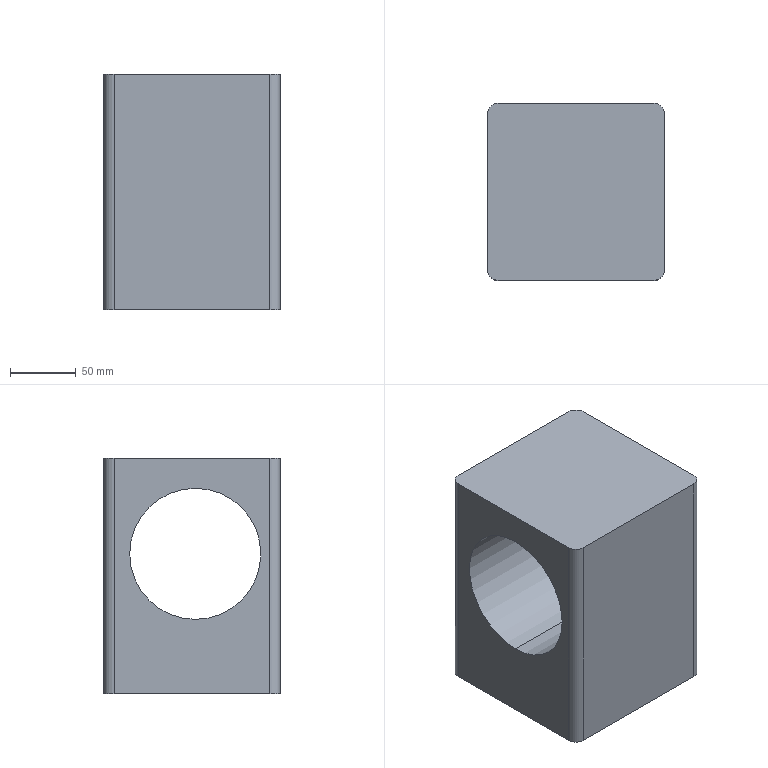Component | SolidWorks | Cam-1 | 1 solid | 12 faces | box 135 x 135 x 180 mm | volume 2209899 mm3 | cylinder 6 | plane 6 | commonest cylinder face diameters 16 x4 100.02 x2
build123d program:
from build123d import *

# Parameters (mm, degrees)
BOSS_EXTRUDE1_DEPTH          = 180
SKETCH1_R                    = 50.01
REPAIR_CAMSHAFTBORE100_DEPTH = 68.5


with BuildPart() as part:
    # Sketch1_2 → Boss-Extrude1 (new body)
    with BuildSketch(Plane.XY.offset(180)):
        with BuildLine():
            Line((59.5, 67.5), (-59.5, 67.5))
            ThreePointArc((-59.5, 67.5), (-65.157, 65.157), (-67.5, 59.5))
            Line((-67.5, 59.5), (-67.5, -59.5))
            ThreePointArc((-67.5, -59.5), (-65.157, -65.157), (-59.5, -67.5))
            Line((-59.5, -67.5), (59.5, -67.5))
            ThreePointArc((59.5, -67.5), (65.157, -65.157), (67.5, -59.5))
            Line((67.5, -59.5), (67.5, 59.5))
            ThreePointArc((67.5, 59.5), (65.157, 65.157), (59.5, 67.5))
        make_face()
    extrude(amount=-BOSS_EXTRUDE1_DEPTH)

    # Sketch1 → Repair_CamshaftBore100 (cut, symmetric)
    with BuildSketch(Plane(origin=(0, 0, 0), x_dir=(1, 0, 0), z_dir=(0, 1, 0))):
        with Locations(Location((-2.5, -106.906, 0), (0, 0, 270))):
            Circle(SKETCH1_R)
    extrude(amount=REPAIR_CAMSHAFTBORE100_DEPTH, both=True, mode=Mode.SUBTRACT)


solid = part.part

# Placed as in the assembly
solid = solid.moved(Location((-505.158, 873.269, 1009.441), (0, 0, 90)))
STEP:
#1=COLOUR_RGB('',0.7922,0.8196,0.9333);
#2=FILL_AREA_STYLE_COLOUR('',#1);
#3=FILL_AREA_STYLE('',(#2));
#4=SURFACE_STYLE_FILL_AREA(#3);
#5=SURFACE_SIDE_STYLE('',(#4));
#6=SURFACE_STYLE_USAGE(.BOTH.,#5);
#7=PRESENTATION_STYLE_ASSIGNMENT((#6));
#8=CARTESIAN_POINT('',(-17.231,34.282,45.92));
#9=VERTEX_POINT('',#8);
#10=CARTESIAN_POINT('',(-17.231,34.282,41.982));
#11=VERTEX_POINT('',#10);
#12=CARTESIAN_POINT('',(-17.231,34.282,43.951));
#13=DIRECTION('',(1.,0.,0.));
#14=DIRECTION('',(0.,0.,-1.));
#15=AXIS2_PLACEMENT_3D('',#12,#13,#14);
#16=CIRCLE('',#15,1.969);
#17=EDGE_CURVE('',#9,#11,#16,.T.);
#18=ORIENTED_EDGE('',*,*,#17,.T.);
#19=CARTESIAN_POINT('',(-22.546,34.282,41.982));
#20=VERTEX_POINT('',#19);
#21=CARTESIAN_POINT('',(-17.191,34.282,41.982));
#22=DIRECTION('',(-1.,0.,0.));
#23=VECTOR('',#22,39.37);
#24=LINE('',#21,#23);
#25=EDGE_CURVE('',#11,#20,#24,.T.);
#26=ORIENTED_EDGE('',*,*,#25,.T.);
#27=CARTESIAN_POINT('',(-22.546,34.282,45.92));
#28=VERTEX_POINT('',#27);
#29=CARTESIAN_POINT('',(-22.546,34.282,43.951));
#30=DIRECTION('',(-1.,0.,0.));
#31=DIRECTION('',(0.,0.,1.));
#32=AXIS2_PLACEMENT_3D('',#29,#30,#31);
#33=CIRCLE('',#32,1.969);
#34=EDGE_CURVE('',#20,#28,#33,.T.);
#35=ORIENTED_EDGE('',*,*,#34,.T.);
#36=CARTESIAN_POINT('',(-17.191,34.282,45.92));
#37=DIRECTION('',(-1.,0.,0.));
#38=VECTOR('',#37,39.37);
#39=LINE('',#36,#38);
#40=EDGE_CURVE('',#9,#28,#39,.T.);
#41=ORIENTED_EDGE('',*,*,#40,.F.);
#42=EDGE_LOOP('',(#18,#26,#35,#41));
#43=FACE_OUTER_BOUND('',#42,.T.);
#44=CARTESIAN_POINT('',(-17.191,34.282,43.951));
#45=DIRECTION('',(-1.,0.,0.));
#46=DIRECTION('',(0.,0.,1.));
#47=AXIS2_PLACEMENT_3D('',#44,#45,#46);
#48=CYLINDRICAL_SURFACE('',#47,1.969);
#49=ADVANCED_FACE('',(#43),#48,.F.);
#50=CARTESIAN_POINT('',(-22.231,37.038,46.828));
#51=VERTEX_POINT('',#50);
#52=CARTESIAN_POINT('',(-22.546,36.723,46.828));
#53=VERTEX_POINT('',#52);
#54=CARTESIAN_POINT('',(-22.231,36.723,46.828));
#55=DIRECTION('',(0.,0.,1.));
#56=DIRECTION('',(0.,1.,0.));
#57=AXIS2_PLACEMENT_3D('',#54,#55,#56);
#58=CIRCLE('',#57,0.315);
#59=EDGE_CURVE('',#51,#53,#58,.T.);
#60=ORIENTED_EDGE('',*,*,#59,.F.);
#61=CARTESIAN_POINT('',(-22.231,37.038,39.742));
#62=VERTEX_POINT('',#61);
#63=CARTESIAN_POINT('',(-22.231,37.038,39.742));
#64=DIRECTION('',(0.,0.,1.));
#65=VECTOR('',#64,39.37);
#66=LINE('',#63,#65);
#67=EDGE_CURVE('',#62,#51,#66,.T.);
#68=ORIENTED_EDGE('',*,*,#67,.F.);
#69=CARTESIAN_POINT('',(-22.546,36.723,39.742));
#70=VERTEX_POINT('',#69);
#71=CARTESIAN_POINT('',(-22.231,36.723,39.742));
#72=DIRECTION('',(0.,0.,1.));
#73=DIRECTION('',(0.,1.,0.));
#74=AXIS2_PLACEMENT_3D('',#71,#72,#73);
#75=CIRCLE('',#74,0.315);
#76=EDGE_CURVE('',#62,#70,#75,.T.);
#77=ORIENTED_EDGE('',*,*,#76,.T.);
#78=CARTESIAN_POINT('',(-22.546,36.723,39.742));
#79=DIRECTION('',(0.,0.,1.));
#80=VECTOR('',#79,39.37);
#81=LINE('',#78,#80);
#82=EDGE_CURVE('',#70,#53,#81,.T.);
#83=ORIENTED_EDGE('',*,*,#82,.T.);
#84=EDGE_LOOP('',(#60,#68,#77,#83));
#85=FACE_OUTER_BOUND('',#84,.T.);
#86=CARTESIAN_POINT('',(-22.231,36.723,39.742));
#87=DIRECTION('',(0.,0.,1.));
#88=DIRECTION('',(0.,1.,0.));
#89=AXIS2_PLACEMENT_3D('',#86,#87,#88);
#90=CYLINDRICAL_SURFACE('',#89,0.315);
#91=ADVANCED_FACE('',(#85),#90,.T.);
#92=CARTESIAN_POINT('',(-17.546,37.038,46.828));
#93=VERTEX_POINT('',#92);
#94=CARTESIAN_POINT('',(-17.546,37.038,46.828));
#95=DIRECTION('',(-1.,0.,0.));
#96=VECTOR('',#95,39.37);
#97=LINE('',#94,#96);
#98=EDGE_CURVE('',#93,#51,#97,.T.);
#99=ORIENTED_EDGE('',*,*,#98,.F.);
#100=CARTESIAN_POINT('',(-17.546,37.038,39.742));
#101=VERTEX_POINT('',#100);
#102=CARTESIAN_POINT('',(-17.546,37.038,39.742));
#103=DIRECTION('',(0.,0.,1.));
#104=VECTOR('',#103,39.37);
#105=LINE('',#102,#104);
#106=EDGE_CURVE('',#101,#93,#105,.T.);
#107=ORIENTED_EDGE('',*,*,#106,.F.);
#108=CARTESIAN_POINT('',(-17.546,37.038,39.742));
#109=DIRECTION('',(-1.,0.,0.));
#110=VECTOR('',#109,39.37);
#111=LINE('',#108,#110);
#112=EDGE_CURVE('',#101,#62,#111,.T.);
#113=ORIENTED_EDGE('',*,*,#112,.T.);
#114=ORIENTED_EDGE('',*,*,#67,.T.);
#115=EDGE_LOOP('',(#99,#107,#113,#114));
#116=FACE_OUTER_BOUND('',#115,.T.);
#117=CARTESIAN_POINT('',(-17.546,37.038,39.742));
#118=DIRECTION('',(0.,1.,0.));
#119=DIRECTION('',(0.,0.,-1.));
#120=AXIS2_PLACEMENT_3D('',#117,#118,#119);
#121=PLANE('',#120);
#122=ADVANCED_FACE('',(#116),#121,.T.);
#123=CARTESIAN_POINT('',(-17.231,36.723,46.828));
#124=VERTEX_POINT('',#123);
#125=CARTESIAN_POINT('',(-17.546,36.723,46.828));
#126=DIRECTION('',(0.,0.,1.));
#127=DIRECTION('',(0.,1.,0.));
#128=AXIS2_PLACEMENT_3D('',#125,#126,#127);
#129=CIRCLE('',#128,0.315);
#130=EDGE_CURVE('',#124,#93,#129,.T.);
#131=ORIENTED_EDGE('',*,*,#130,.F.);
#132=CARTESIAN_POINT('',(-17.231,36.723,39.742));
#133=VERTEX_POINT('',#132);
#134=CARTESIAN_POINT('',(-17.231,36.723,39.742));
#135=DIRECTION('',(0.,0.,1.));
#136=VECTOR('',#135,39.37);
#137=LINE('',#134,#136);
#138=EDGE_CURVE('',#133,#124,#137,.T.);
#139=ORIENTED_EDGE('',*,*,#138,.F.);
#140=CARTESIAN_POINT('',(-17.546,36.723,39.742));
#141=DIRECTION('',(0.,0.,1.));
#142=DIRECTION('',(0.,1.,0.));
#143=AXIS2_PLACEMENT_3D('',#140,#141,#142);
#144=CIRCLE('',#143,0.315);
#145=EDGE_CURVE('',#133,#101,#144,.T.);
#146=ORIENTED_EDGE('',*,*,#145,.T.);
#147=ORIENTED_EDGE('',*,*,#106,.T.);
#148=EDGE_LOOP('',(#131,#139,#146,#147));
#149=FACE_OUTER_BOUND('',#148,.T.);
#150=CARTESIAN_POINT('',(-17.546,36.723,39.742));
#151=DIRECTION('',(0.,0.,1.));
#152=DIRECTION('',(0.,1.,0.));
#153=AXIS2_PLACEMENT_3D('',#150,#151,#152);
#154=CYLINDRICAL_SURFACE('',#153,0.315);
#155=ADVANCED_FACE('',(#149),#154,.T.);
#156=ORIENTED_EDGE('',*,*,#17,.F.);
#157=CARTESIAN_POINT('',(-17.231,34.282,43.951));
#158=DIRECTION('',(1.,0.,0.));
#159=DIRECTION('',(0.,0.,-1.));
#160=AXIS2_PLACEMENT_3D('',#157,#158,#159);
#161=CIRCLE('',#160,1.969);
#162=EDGE_CURVE('',#11,#9,#161,.T.);
#163=ORIENTED_EDGE('',*,*,#162,.F.);
#164=EDGE_LOOP('',(#156,#163));
#165=FACE_BOUND('',#164,.T.);
#166=CARTESIAN_POINT('',(-17.231,32.038,46.828));
#167=VERTEX_POINT('',#166);
#168=CARTESIAN_POINT('',(-17.231,32.038,46.828));
#169=DIRECTION('',(0.,1.,0.));
#170=VECTOR('',#169,39.37);
#171=LINE('',#168,#170);
#172=EDGE_CURVE('',#167,#124,#171,.T.);
#173=ORIENTED_EDGE('',*,*,#172,.F.);
#174=CARTESIAN_POINT('',(-17.231,32.038,39.742));
#175=VERTEX_POINT('',#174);
#176=CARTESIAN_POINT('',(-17.231,32.038,39.742));
#177=DIRECTION('',(0.,0.,1.));
#178=VECTOR('',#177,39.37);
#179=LINE('',#176,#178);
#180=EDGE_CURVE('',#175,#167,#179,.T.);
#181=ORIENTED_EDGE('',*,*,#180,.F.);
#182=CARTESIAN_POINT('',(-17.231,32.038,39.742));
#183=DIRECTION('',(0.,1.,0.));
#184=VECTOR('',#183,39.37);
#185=LINE('',#182,#184);
#186=EDGE_CURVE('',#175,#133,#185,.T.);
#187=ORIENTED_EDGE('',*,*,#186,.T.);
#188=ORIENTED_EDGE('',*,*,#138,.T.);
#189=EDGE_LOOP('',(#173,#181,#187,#188));
#190=FACE_OUTER_BOUND('',#189,.T.);
#191=CARTESIAN_POINT('',(-17.231,32.038,39.742));
#192=DIRECTION('',(1.,0.,0.));
#193=DIRECTION('',(0.,0.,-1.));
#194=AXIS2_PLACEMENT_3D('',#191,#192,#193);
#195=PLANE('',#194);
#196=ADVANCED_FACE('',(#165,#190),#195,.T.);
#197=CARTESIAN_POINT('',(-17.546,31.723,46.828));
#198=VERTEX_POINT('',#197);
#199=CARTESIAN_POINT('',(-17.546,32.038,46.828));
#200=DIRECTION('',(0.,0.,1.));
#201=DIRECTION('',(0.,1.,0.));
#202=AXIS2_PLACEMENT_3D('',#199,#200,#201);
#203=CIRCLE('',#202,0.315);
#204=EDGE_CURVE('',#198,#167,#203,.T.);
#205=ORIENTED_EDGE('',*,*,#204,.F.);
#206=CARTESIAN_POINT('',(-17.546,31.723,39.742));
#207=VERTEX_POINT('',#206);
#208=CARTESIAN_POINT('',(-17.546,31.723,39.742));
#209=DIRECTION('',(0.,0.,1.));
#210=VECTOR('',#209,39.37);
#211=LINE('',#208,#210);
#212=EDGE_CURVE('',#207,#198,#211,.T.);
#213=ORIENTED_EDGE('',*,*,#212,.F.);
#214=CARTESIAN_POINT('',(-17.546,32.038,39.742));
#215=DIRECTION('',(0.,0.,1.));
#216=DIRECTION('',(0.,1.,0.));
#217=AXIS2_PLACEMENT_3D('',#214,#215,#216);
#218=CIRCLE('',#217,0.315);
#219=EDGE_CURVE('',#207,#175,#218,.T.);
#220=ORIENTED_EDGE('',*,*,#219,.T.);
#221=ORIENTED_EDGE('',*,*,#180,.T.);
#222=EDGE_LOOP('',(#205,#213,#220,#221));
#223=FACE_OUTER_BOUND('',#222,.T.);
#224=CARTESIAN_POINT('',(-17.546,32.038,39.742));
#225=DIRECTION('',(0.,0.,1.));
#226=DIRECTION('',(0.,1.,0.));
#227=AXIS2_PLACEMENT_3D('',#224,#225,#226);
#228=CYLINDRICAL_SURFACE('',#227,0.315);
#229=ADVANCED_FACE('',(#223),#228,.T.);
#230=CARTESIAN_POINT('',(-22.231,31.723,46.828));
#231=VERTEX_POINT('',#230);
#232=CARTESIAN_POINT('',(-22.231,31.723,46.828));
#233=DIRECTION('',(1.,0.,0.));
#234=VECTOR('',#233,39.37);
#235=LINE('',#232,#234);
#236=EDGE_CURVE('',#231,#198,#235,.T.);
#237=ORIENTED_EDGE('',*,*,#236,.F.);
#238=CARTESIAN_POINT('',(-22.231,31.723,39.742));
#239=VERTEX_POINT('',#238);
#240=CARTESIAN_POINT('',(-22.231,31.723,39.742));
#241=DIRECTION('',(0.,0.,1.));
#242=VECTOR('',#241,39.37);
#243=LINE('',#240,#242);
#244=EDGE_CURVE('',#239,#231,#243,.T.);
#245=ORIENTED_EDGE('',*,*,#244,.F.);
#246=CARTESIAN_POINT('',(-22.231,31.723,39.742));
#247=DIRECTION('',(1.,0.,0.));
#248=VECTOR('',#247,39.37);
#249=LINE('',#246,#248);
#250=EDGE_CURVE('',#239,#207,#249,.T.);
#251=ORIENTED_EDGE('',*,*,#250,.T.);
#252=ORIENTED_EDGE('',*,*,#212,.T.);
#253=EDGE_LOOP('',(#237,#245,#251,#252));
#254=FACE_OUTER_BOUND('',#253,.T.);
#255=CARTESIAN_POINT('',(-22.231,31.723,39.742));
#256=DIRECTION('',(0.,-1.,0.));
#257=DIRECTION('',(0.,0.,1.));
#258=AXIS2_PLACEMENT_3D('',#255,#256,#257);
#259=PLANE('',#258);
#260=ADVANCED_FACE('',(#254),#259,.T.);
#261=CARTESIAN_POINT('',(-22.546,32.038,46.828));
#262=VERTEX_POINT('',#261);
#263=CARTESIAN_POINT('',(-22.231,32.038,46.828));
#264=DIRECTION('',(0.,0.,1.));
#265=DIRECTION('',(0.,1.,0.));
#266=AXIS2_PLACEMENT_3D('',#263,#264,#265);
#267=CIRCLE('',#266,0.315);
#268=EDGE_CURVE('',#262,#231,#267,.T.);
#269=ORIENTED_EDGE('',*,*,#268,.F.);
#270=CARTESIAN_POINT('',(-22.546,32.038,39.742));
#271=VERTEX_POINT('',#270);
#272=CARTESIAN_POINT('',(-22.546,32.038,39.742));
#273=DIRECTION('',(0.,0.,1.));
#274=VECTOR('',#273,39.37);
#275=LINE('',#272,#274);
#276=EDGE_CURVE('',#271,#262,#275,.T.);
#277=ORIENTED_EDGE('',*,*,#276,.F.);
#278=CARTESIAN_POINT('',(-22.231,32.038,39.742));
#279=DIRECTION('',(0.,0.,1.));
#280=DIRECTION('',(0.,1.,0.));
#281=AXIS2_PLACEMENT_3D('',#278,#279,#280);
#282=CIRCLE('',#281,0.315);
#283=EDGE_CURVE('',#271,#239,#282,.T.);
#284=ORIENTED_EDGE('',*,*,#283,.T.);
#285=ORIENTED_EDGE('',*,*,#244,.T.);
#286=EDGE_LOOP('',(#269,#277,#284,#285));
#287=FACE_OUTER_BOUND('',#286,.T.);
#288=CARTESIAN_POINT('',(-22.231,32.038,39.742));
#289=DIRECTION('',(0.,0.,1.));
#290=DIRECTION('',(0.,1.,0.));
#291=AXIS2_PLACEMENT_3D('',#288,#289,#290);
#292=CYLINDRICAL_SURFACE('',#291,0.315);
#293=ADVANCED_FACE('',(#287),#292,.T.);
#294=CARTESIAN_POINT('',(-22.546,34.282,43.951));
#295=DIRECTION('',(-1.,0.,0.));
#296=DIRECTION('',(0.,0.,1.));
#297=AXIS2_PLACEMENT_3D('',#294,#295,#296);
#298=CIRCLE('',#297,1.969);
#299=EDGE_CURVE('',#28,#20,#298,.T.);
#300=ORIENTED_EDGE('',*,*,#299,.F.);
#301=ORIENTED_EDGE('',*,*,#34,.F.);
#302=EDGE_LOOP('',(#300,#301));
#303=FACE_BOUND('',#302,.T.);
#304=CARTESIAN_POINT('',(-22.546,36.723,46.828));
#305=DIRECTION('',(0.,-1.,0.));
#306=VECTOR('',#305,39.37);
#307=LINE('',#304,#306);
#308=EDGE_CURVE('',#53,#262,#307,.T.);
#309=ORIENTED_EDGE('',*,*,#308,.F.);
#310=ORIENTED_EDGE('',*,*,#82,.F.);
#311=CARTESIAN_POINT('',(-22.546,36.723,39.742));
#312=DIRECTION('',(0.,-1.,0.));
#313=VECTOR('',#312,39.37);
#314=LINE('',#311,#313);
#315=EDGE_CURVE('',#70,#271,#314,.T.);
#316=ORIENTED_EDGE('',*,*,#315,.T.);
#317=ORIENTED_EDGE('',*,*,#276,.T.);
#318=EDGE_LOOP('',(#309,#310,#316,#317));
#319=FACE_OUTER_BOUND('',#318,.T.);
#320=CARTESIAN_POINT('',(-22.546,36.723,39.742));
#321=DIRECTION('',(-1.,0.,0.));
#322=DIRECTION('',(0.,0.,1.));
#323=AXIS2_PLACEMENT_3D('',#320,#321,#322);
#324=PLANE('',#323);
#325=ADVANCED_FACE('',(#303,#319),#324,.T.);
#326=ORIENTED_EDGE('',*,*,#76,.F.);
#327=ORIENTED_EDGE('',*,*,#112,.F.);
#328=ORIENTED_EDGE('',*,*,#145,.F.);
#329=ORIENTED_EDGE('',*,*,#186,.F.);
#330=ORIENTED_EDGE('',*,*,#219,.F.);
#331=ORIENTED_EDGE('',*,*,#250,.F.);
#332=ORIENTED_EDGE('',*,*,#283,.F.);
#333=ORIENTED_EDGE('',*,*,#315,.F.);
#334=EDGE_LOOP('',(#326,#327,#328,#329,#330,#331,#332,#333));
#335=FACE_OUTER_BOUND('',#334,.T.);
#336=CARTESIAN_POINT('',(-22.231,36.723,39.742));
#337=DIRECTION('',(0.,0.,1.));
#338=DIRECTION('',(0.,1.,0.));
#339=AXIS2_PLACEMENT_3D('',#336,#337,#338);
#340=PLANE('',#339);
#341=ADVANCED_FACE('',(#335),#340,.F.);
#342=ORIENTED_EDGE('',*,*,#59,.T.);
#343=ORIENTED_EDGE('',*,*,#308,.T.);
#344=ORIENTED_EDGE('',*,*,#268,.T.);
#345=ORIENTED_EDGE('',*,*,#236,.T.);
#346=ORIENTED_EDGE('',*,*,#204,.T.);
#347=ORIENTED_EDGE('',*,*,#172,.T.);
#348=ORIENTED_EDGE('',*,*,#130,.T.);
#349=ORIENTED_EDGE('',*,*,#98,.T.);
#350=EDGE_LOOP('',(#342,#343,#344,#345,#346,#347,#348,#349));
#351=FACE_OUTER_BOUND('',#350,.T.);
#352=CARTESIAN_POINT('',(-22.231,36.723,46.828));
#353=DIRECTION('',(0.,0.,1.));
#354=DIRECTION('',(0.,1.,0.));
#355=AXIS2_PLACEMENT_3D('',#352,#353,#354);
#356=PLANE('',#355);
#357=ADVANCED_FACE('',(#351),#356,.T.);
#358=ORIENTED_EDGE('',*,*,#25,.F.);
#359=ORIENTED_EDGE('',*,*,#162,.T.);
#360=ORIENTED_EDGE('',*,*,#40,.T.);
#361=ORIENTED_EDGE('',*,*,#299,.T.);
#362=EDGE_LOOP('',(#358,#359,#360,#361));
#363=FACE_OUTER_BOUND('',#362,.T.);
#364=CARTESIAN_POINT('',(-17.191,34.282,43.951));
#365=DIRECTION('',(-1.,0.,0.));
#366=DIRECTION('',(0.,0.,1.));
#367=AXIS2_PLACEMENT_3D('',#364,#365,#366);
#368=CYLINDRICAL_SURFACE('',#367,1.969);
#369=ADVANCED_FACE('',(#363),#368,.F.);
#370=CLOSED_SHELL('',(#49,#91,#122,#155,#196,#229,#260,#293,#325,#341,#357,#369));
#371=MANIFOLD_SOLID_BREP('',#370);
#372=STYLED_ITEM('',(#7),#371);
#373=PRESENTATION_LAYER_ASSIGNMENT('','',(#372));
#374=CARTESIAN_POINT('',(0.,0.,0.));
#375=DIRECTION('',(0.,0.,1.));
#376=DIRECTION('',(1.,0.,0.));
#377=AXIS2_PLACEMENT_3D('',#374,#375,#376);
#378=(LENGTH_UNIT()NAMED_UNIT(*)SI_UNIT($,.METRE.));
#379=LENGTH_MEASURE_WITH_UNIT(LENGTH_MEASURE(0.0254),#378);
#380=DIMENSIONAL_EXPONENTS(1.,0.,0.,0.,0.,0.,0.);
#381=(CONVERSION_BASED_UNIT('',#379)LENGTH_UNIT()NAMED_UNIT(#380));
#382=UNCERTAINTY_MEASURE_WITH_UNIT(LENGTH_MEASURE(0.00001),#381,'','');
#383=(NAMED_UNIT(*)PLANE_ANGLE_UNIT()SI_UNIT($,.RADIAN.));
#384=(NAMED_UNIT(*)SI_UNIT($,.STERADIAN.)SOLID_ANGLE_UNIT());
#385=(GEOMETRIC_REPRESENTATION_CONTEXT(3)GLOBAL_UNCERTAINTY_ASSIGNED_CONTEXT((#382))GLOBAL_UNIT_ASSIGNED_CONTEXT((#381,#383,#384))REPRESENTATION_CONTEXT('',''));
#386=ADVANCED_BREP_SHAPE_REPRESENTATION('',(#371,#377),#385);
#387=(LENGTH_UNIT()NAMED_UNIT(*)SI_UNIT($,.METRE.));
#388=LENGTH_MEASURE_WITH_UNIT(LENGTH_MEASURE(0.0254),#387);
#389=DIMENSIONAL_EXPONENTS(1.,0.,0.,0.,0.,0.,0.);
#390=(CONVERSION_BASED_UNIT('',#388)LENGTH_UNIT()NAMED_UNIT(#389));
#391=UNCERTAINTY_MEASURE_WITH_UNIT(LENGTH_MEASURE(0.00001),#390,'','');
#392=(NAMED_UNIT(*)PLANE_ANGLE_UNIT()SI_UNIT($,.RADIAN.));
#393=(NAMED_UNIT(*)SI_UNIT($,.STERADIAN.)SOLID_ANGLE_UNIT());
#394=(GEOMETRIC_REPRESENTATION_CONTEXT(3)GLOBAL_UNCERTAINTY_ASSIGNED_CONTEXT((#391))GLOBAL_UNIT_ASSIGNED_CONTEXT((#390,#392,#393))REPRESENTATION_CONTEXT('',''));
#395=MECHANICAL_DESIGN_GEOMETRIC_PRESENTATION_REPRESENTATION('',(#372),#394);